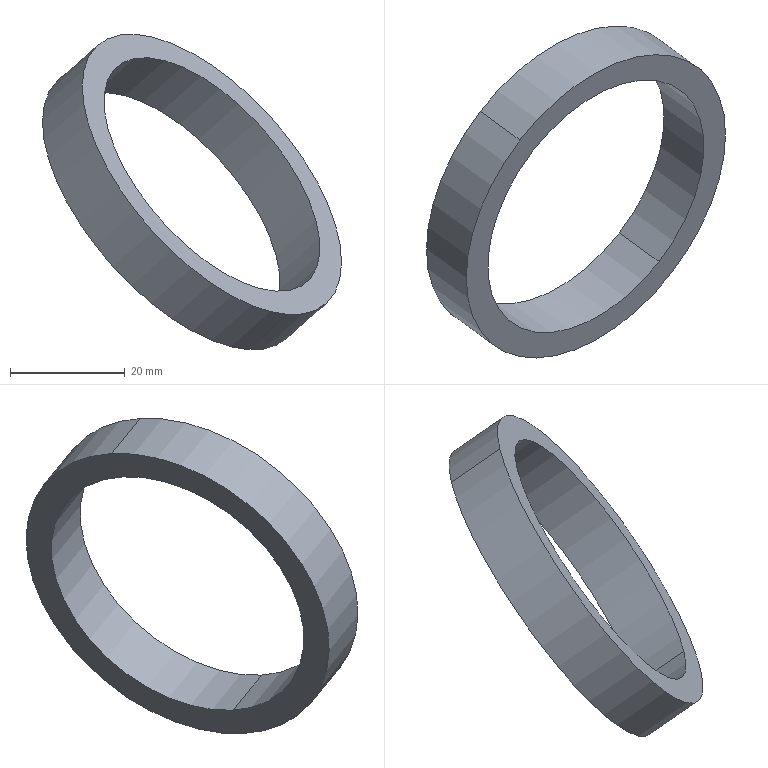Component | SolidWorks | Gasket-1 | 1 solid | 6 faces | box 52.04 x 57.76 x 54.91 mm | volume 9071 mm3 | cylinder 4 | plane 2 | commonest cylinder face diameters 50 x2 60 x2 | material Copper
build123d program:
from build123d import *

# Parameters (mm, degrees)
SKETCH1_R           = 30
SKETCH1_R_2         = 25
BOSS_EXTRUDE1_DEPTH = 10.5


with BuildPart() as part:
    # Sketch1 → Boss-Extrude1 (new body)
    with BuildSketch(Plane(origin=(0, 0, 0), x_dir=(1, 0, 0), z_dir=(0, 1, 0))):
        with Locations(Location((0, 0, 0), (0, 0, 90))):
            Circle(SKETCH1_R)
        with Locations(Location((0, 0, 0), (0, 0, 90))):
            Circle(SKETCH1_R_2, mode=Mode.SUBTRACT)
    extrude(amount=BOSS_EXTRUDE1_DEPTH)


solid = part.part

# Placed as in the assembly
solid = solid.moved(Location((188.537, -1911.326, 439.699), (-120.831, 47.011, -104.803)))
STEP:
#1=CARTESIAN_POINT('',(7.856,-75.626,16.512));
#2=VERTEX_POINT('',#1);
#3=CARTESIAN_POINT('',(6.99,-74.872,18.11));
#4=VERTEX_POINT('',#3);
#5=CARTESIAN_POINT('',(7.423,-75.249,17.311));
#6=DIRECTION('',(-0.6592,0.4763,-0.5818));
#7=DIRECTION('',(-0.4398,0.3834,0.8122));
#8=AXIS2_PLACEMENT_3D('',#5,#6,#7);
#9=CIRCLE('',#8,0.9843);
#10=EDGE_CURVE('',#2,#4,#9,.T.);
#11=ORIENTED_EDGE('',*,*,#10,.T.);
#12=CARTESIAN_POINT('',(7.262,-75.069,18.351));
#13=VERTEX_POINT('',#12);
#14=CARTESIAN_POINT('',(6.99,-74.872,18.11));
#15=DIRECTION('',(0.6592,-0.4763,0.5818));
#16=VECTOR('',#15,39.37);
#17=LINE('',#14,#16);
#18=EDGE_CURVE('',#4,#13,#17,.T.);
#19=ORIENTED_EDGE('',*,*,#18,.T.);
#20=CARTESIAN_POINT('',(8.128,-75.823,16.752));
#21=VERTEX_POINT('',#20);
#22=CARTESIAN_POINT('',(7.695,-75.446,17.551));
#23=DIRECTION('',(-0.6592,0.4763,-0.5818));
#24=DIRECTION('',(-0.4398,0.3834,0.8122));
#25=AXIS2_PLACEMENT_3D('',#22,#23,#24);
#26=CIRCLE('',#25,0.9843);
#27=EDGE_CURVE('',#21,#13,#26,.T.);
#28=ORIENTED_EDGE('',*,*,#27,.F.);
#29=CARTESIAN_POINT('',(7.856,-75.626,16.512));
#30=DIRECTION('',(0.6592,-0.4763,0.5818));
#31=VECTOR('',#30,39.37);
#32=LINE('',#29,#31);
#33=EDGE_CURVE('',#2,#21,#32,.T.);
#34=ORIENTED_EDGE('',*,*,#33,.F.);
#35=EDGE_LOOP('',(#11,#19,#28,#34));
#36=FACE_OUTER_BOUND('',#35,.T.);
#37=CARTESIAN_POINT('',(7.423,-75.249,17.311));
#38=DIRECTION('',(0.6592,-0.4763,0.5818));
#39=DIRECTION('',(0.4398,-0.3834,-0.8122));
#40=AXIS2_PLACEMENT_3D('',#37,#38,#39);
#41=CYLINDRICAL_SURFACE('',#40,0.9843);
#42=ADVANCED_FACE('',(#36),#41,.F.);
#43=CARTESIAN_POINT('',(6.903,-74.796,18.27));
#44=VERTEX_POINT('',#43);
#45=CARTESIAN_POINT('',(7.942,-75.702,16.352));
#46=VERTEX_POINT('',#45);
#47=CARTESIAN_POINT('',(7.423,-75.249,17.311));
#48=DIRECTION('',(-0.6592,0.4763,-0.5818));
#49=DIRECTION('',(-0.4398,0.3834,0.8122));
#50=AXIS2_PLACEMENT_3D('',#47,#48,#49);
#51=CIRCLE('',#50,1.181);
#52=EDGE_CURVE('',#44,#46,#51,.T.);
#53=ORIENTED_EDGE('',*,*,#52,.F.);
#54=CARTESIAN_POINT('',(7.176,-74.993,18.511));
#55=VERTEX_POINT('',#54);
#56=CARTESIAN_POINT('',(6.903,-74.796,18.27));
#57=DIRECTION('',(0.6592,-0.4763,0.5818));
#58=VECTOR('',#57,39.37);
#59=LINE('',#56,#58);
#60=EDGE_CURVE('',#44,#55,#59,.T.);
#61=ORIENTED_EDGE('',*,*,#60,.T.);
#62=CARTESIAN_POINT('',(8.215,-75.899,16.592));
#63=VERTEX_POINT('',#62);
#64=CARTESIAN_POINT('',(7.695,-75.446,17.551));
#65=DIRECTION('',(-0.6592,0.4763,-0.5818));
#66=DIRECTION('',(-0.4398,0.3834,0.8122));
#67=AXIS2_PLACEMENT_3D('',#64,#65,#66);
#68=CIRCLE('',#67,1.181);
#69=EDGE_CURVE('',#55,#63,#68,.T.);
#70=ORIENTED_EDGE('',*,*,#69,.T.);
#71=CARTESIAN_POINT('',(7.942,-75.702,16.352));
#72=DIRECTION('',(0.6592,-0.4763,0.5818));
#73=VECTOR('',#72,39.37);
#74=LINE('',#71,#73);
#75=EDGE_CURVE('',#46,#63,#74,.T.);
#76=ORIENTED_EDGE('',*,*,#75,.F.);
#77=EDGE_LOOP('',(#53,#61,#70,#76));
#78=FACE_OUTER_BOUND('',#77,.T.);
#79=CARTESIAN_POINT('',(7.423,-75.249,17.311));
#80=DIRECTION('',(0.6592,-0.4763,0.5818));
#81=DIRECTION('',(0.4398,-0.3834,-0.8122));
#82=AXIS2_PLACEMENT_3D('',#79,#80,#81);
#83=CYLINDRICAL_SURFACE('',#82,1.181);
#84=ADVANCED_FACE('',(#78),#83,.T.);
#85=CARTESIAN_POINT('',(7.423,-75.249,17.311));
#86=DIRECTION('',(-0.6592,0.4763,-0.5818));
#87=DIRECTION('',(-0.4398,0.3834,0.8122));
#88=AXIS2_PLACEMENT_3D('',#85,#86,#87);
#89=CIRCLE('',#88,1.181);
#90=EDGE_CURVE('',#46,#44,#89,.T.);
#91=ORIENTED_EDGE('',*,*,#90,.T.);
#92=ORIENTED_EDGE('',*,*,#52,.T.);
#93=EDGE_LOOP('',(#91,#92));
#94=FACE_OUTER_BOUND('',#93,.T.);
#95=ORIENTED_EDGE('',*,*,#10,.F.);
#96=CARTESIAN_POINT('',(7.423,-75.249,17.311));
#97=DIRECTION('',(-0.6592,0.4763,-0.5818));
#98=DIRECTION('',(-0.4398,0.3834,0.8122));
#99=AXIS2_PLACEMENT_3D('',#96,#97,#98);
#100=CIRCLE('',#99,0.9843);
#101=EDGE_CURVE('',#4,#2,#100,.T.);
#102=ORIENTED_EDGE('',*,*,#101,.F.);
#103=EDGE_LOOP('',(#95,#102));
#104=FACE_BOUND('',#103,.T.);
#105=CARTESIAN_POINT('',(7.423,-75.249,17.311));
#106=DIRECTION('',(-0.6592,0.4763,-0.5818));
#107=DIRECTION('',(-0.4398,0.3834,0.8122));
#108=AXIS2_PLACEMENT_3D('',#105,#106,#107);
#109=PLANE('',#108);
#110=ADVANCED_FACE('',(#94,#104),#109,.T.);
#111=CARTESIAN_POINT('',(7.695,-75.446,17.551));
#112=DIRECTION('',(-0.6592,0.4763,-0.5818));
#113=DIRECTION('',(-0.4398,0.3834,0.8122));
#114=AXIS2_PLACEMENT_3D('',#111,#112,#113);
#115=CIRCLE('',#114,1.181);
#116=EDGE_CURVE('',#63,#55,#115,.T.);
#117=ORIENTED_EDGE('',*,*,#116,.F.);
#118=ORIENTED_EDGE('',*,*,#69,.F.);
#119=EDGE_LOOP('',(#117,#118));
#120=FACE_OUTER_BOUND('',#119,.T.);
#121=ORIENTED_EDGE('',*,*,#27,.T.);
#122=CARTESIAN_POINT('',(7.695,-75.446,17.551));
#123=DIRECTION('',(-0.6592,0.4763,-0.5818));
#124=DIRECTION('',(-0.4398,0.3834,0.8122));
#125=AXIS2_PLACEMENT_3D('',#122,#123,#124);
#126=CIRCLE('',#125,0.9843);
#127=EDGE_CURVE('',#13,#21,#126,.T.);
#128=ORIENTED_EDGE('',*,*,#127,.T.);
#129=EDGE_LOOP('',(#121,#128));
#130=FACE_BOUND('',#129,.T.);
#131=CARTESIAN_POINT('',(7.695,-75.446,17.551));
#132=DIRECTION('',(-0.6592,0.4763,-0.5818));
#133=DIRECTION('',(-0.4398,0.3834,0.8122));
#134=AXIS2_PLACEMENT_3D('',#131,#132,#133);
#135=PLANE('',#134);
#136=ADVANCED_FACE('',(#120,#130),#135,.F.);
#137=ORIENTED_EDGE('',*,*,#60,.F.);
#138=ORIENTED_EDGE('',*,*,#90,.F.);
#139=ORIENTED_EDGE('',*,*,#75,.T.);
#140=ORIENTED_EDGE('',*,*,#116,.T.);
#141=EDGE_LOOP('',(#137,#138,#139,#140));
#142=FACE_OUTER_BOUND('',#141,.T.);
#143=CARTESIAN_POINT('',(7.423,-75.249,17.311));
#144=DIRECTION('',(0.6592,-0.4763,0.5818));
#145=DIRECTION('',(0.4398,-0.3834,-0.8122));
#146=AXIS2_PLACEMENT_3D('',#143,#144,#145);
#147=CYLINDRICAL_SURFACE('',#146,1.181);
#148=ADVANCED_FACE('',(#142),#147,.T.);
#149=ORIENTED_EDGE('',*,*,#18,.F.);
#150=ORIENTED_EDGE('',*,*,#101,.T.);
#151=ORIENTED_EDGE('',*,*,#33,.T.);
#152=ORIENTED_EDGE('',*,*,#127,.F.);
#153=EDGE_LOOP('',(#149,#150,#151,#152));
#154=FACE_OUTER_BOUND('',#153,.T.);
#155=CARTESIAN_POINT('',(7.423,-75.249,17.311));
#156=DIRECTION('',(0.6592,-0.4763,0.5818));
#157=DIRECTION('',(0.4398,-0.3834,-0.8122));
#158=AXIS2_PLACEMENT_3D('',#155,#156,#157);
#159=CYLINDRICAL_SURFACE('',#158,0.9843);
#160=ADVANCED_FACE('',(#154),#159,.F.);
#161=CLOSED_SHELL('',(#42,#84,#110,#136,#148,#160));
#162=MANIFOLD_SOLID_BREP('',#161);
#163=CARTESIAN_POINT('',(0.,0.,0.));
#164=DIRECTION('',(0.,0.,1.));
#165=DIRECTION('',(1.,0.,0.));
#166=AXIS2_PLACEMENT_3D('',#163,#164,#165);
#167=(LENGTH_UNIT()NAMED_UNIT(*)SI_UNIT($,.METRE.));
#168=LENGTH_MEASURE_WITH_UNIT(LENGTH_MEASURE(0.0254),#167);
#169=DIMENSIONAL_EXPONENTS(1.,0.,0.,0.,0.,0.,0.);
#170=(CONVERSION_BASED_UNIT('',#168)LENGTH_UNIT()NAMED_UNIT(#169));
#171=UNCERTAINTY_MEASURE_WITH_UNIT(LENGTH_MEASURE(0.00001),#170,'','');
#172=(NAMED_UNIT(*)PLANE_ANGLE_UNIT()SI_UNIT($,.RADIAN.));
#173=(NAMED_UNIT(*)SI_UNIT($,.STERADIAN.)SOLID_ANGLE_UNIT());
#174=(GEOMETRIC_REPRESENTATION_CONTEXT(3)GLOBAL_UNCERTAINTY_ASSIGNED_CONTEXT((#171))GLOBAL_UNIT_ASSIGNED_CONTEXT((#170,#172,#173))REPRESENTATION_CONTEXT('',''));
#175=ADVANCED_BREP_SHAPE_REPRESENTATION('',(#162,#166),#174);
#176=COLOUR_RGB('',0.7922,0.8196,0.9333);
#177=FILL_AREA_STYLE_COLOUR('',#176);
#178=FILL_AREA_STYLE('',(#177));
#179=SURFACE_STYLE_FILL_AREA(#178);
#180=SURFACE_SIDE_STYLE('',(#179));
#181=SURFACE_STYLE_USAGE(.BOTH.,#180);
#182=PRESENTATION_STYLE_ASSIGNMENT((#181));
#183=STYLED_ITEM('',(#182),#162);
#184=(LENGTH_UNIT()NAMED_UNIT(*)SI_UNIT($,.METRE.));
#185=LENGTH_MEASURE_WITH_UNIT(LENGTH_MEASURE(0.0254),#184);
#186=DIMENSIONAL_EXPONENTS(1.,0.,0.,0.,0.,0.,0.);
#187=(CONVERSION_BASED_UNIT('',#185)LENGTH_UNIT()NAMED_UNIT(#186));
#188=UNCERTAINTY_MEASURE_WITH_UNIT(LENGTH_MEASURE(0.00001),#187,'','');
#189=(NAMED_UNIT(*)PLANE_ANGLE_UNIT()SI_UNIT($,.RADIAN.));
#190=(NAMED_UNIT(*)SI_UNIT($,.STERADIAN.)SOLID_ANGLE_UNIT());
#191=(GEOMETRIC_REPRESENTATION_CONTEXT(3)GLOBAL_UNCERTAINTY_ASSIGNED_CONTEXT((#188))GLOBAL_UNIT_ASSIGNED_CONTEXT((#187,#189,#190))REPRESENTATION_CONTEXT('',''));
#192=MECHANICAL_DESIGN_GEOMETRIC_PRESENTATION_REPRESENTATION('',(#183),#191);
#193=PRESENTATION_LAYER_ASSIGNMENT('','',(#183));